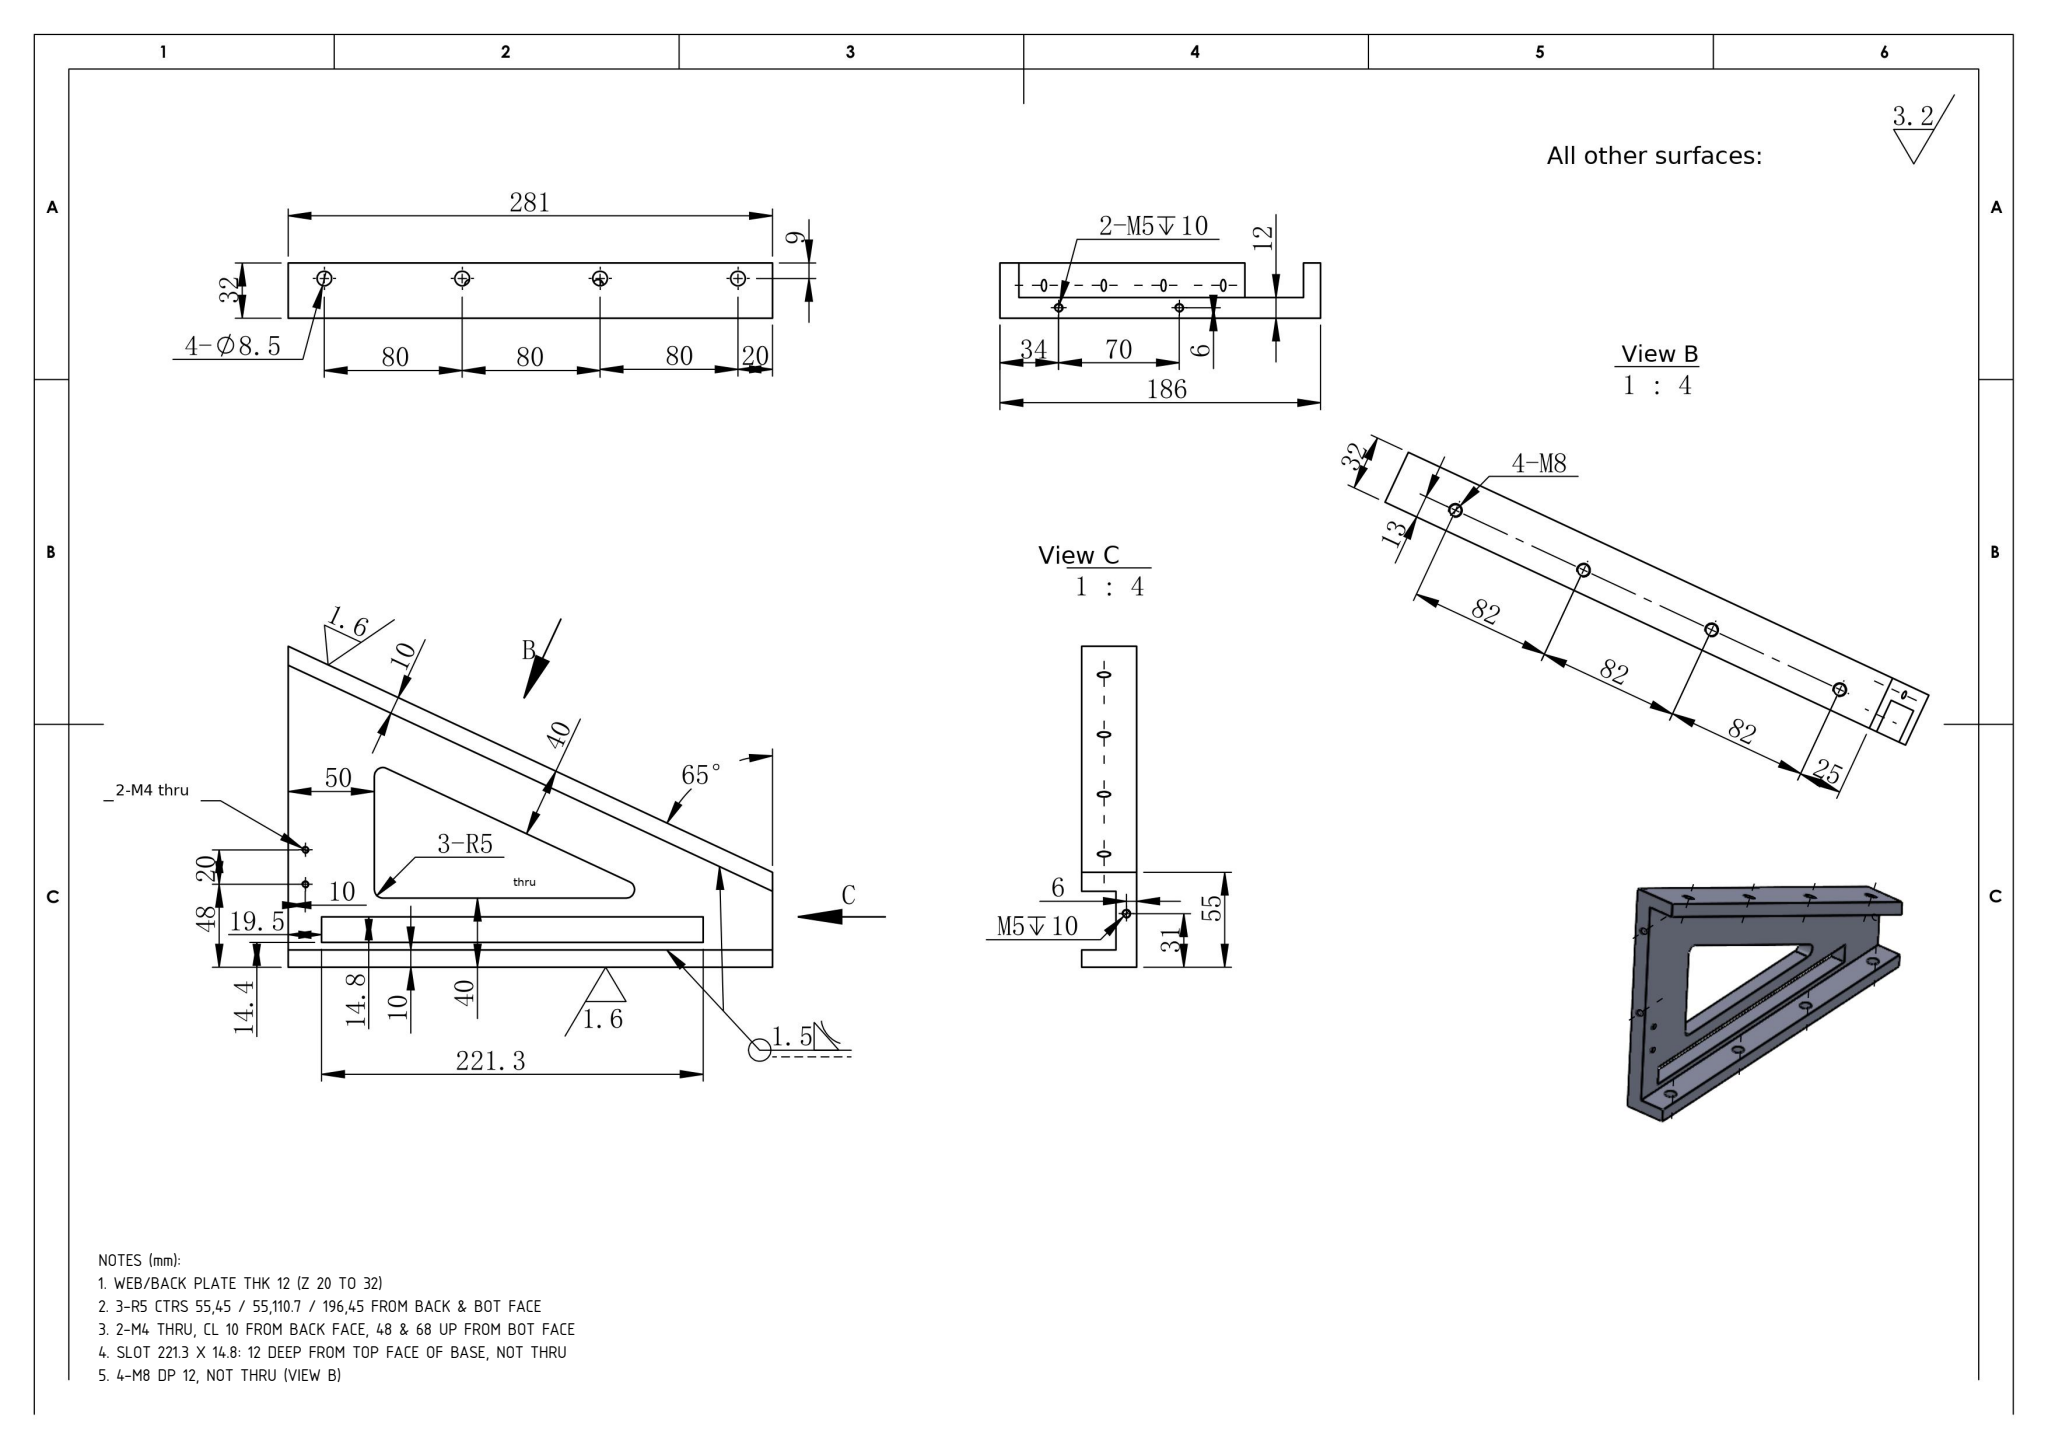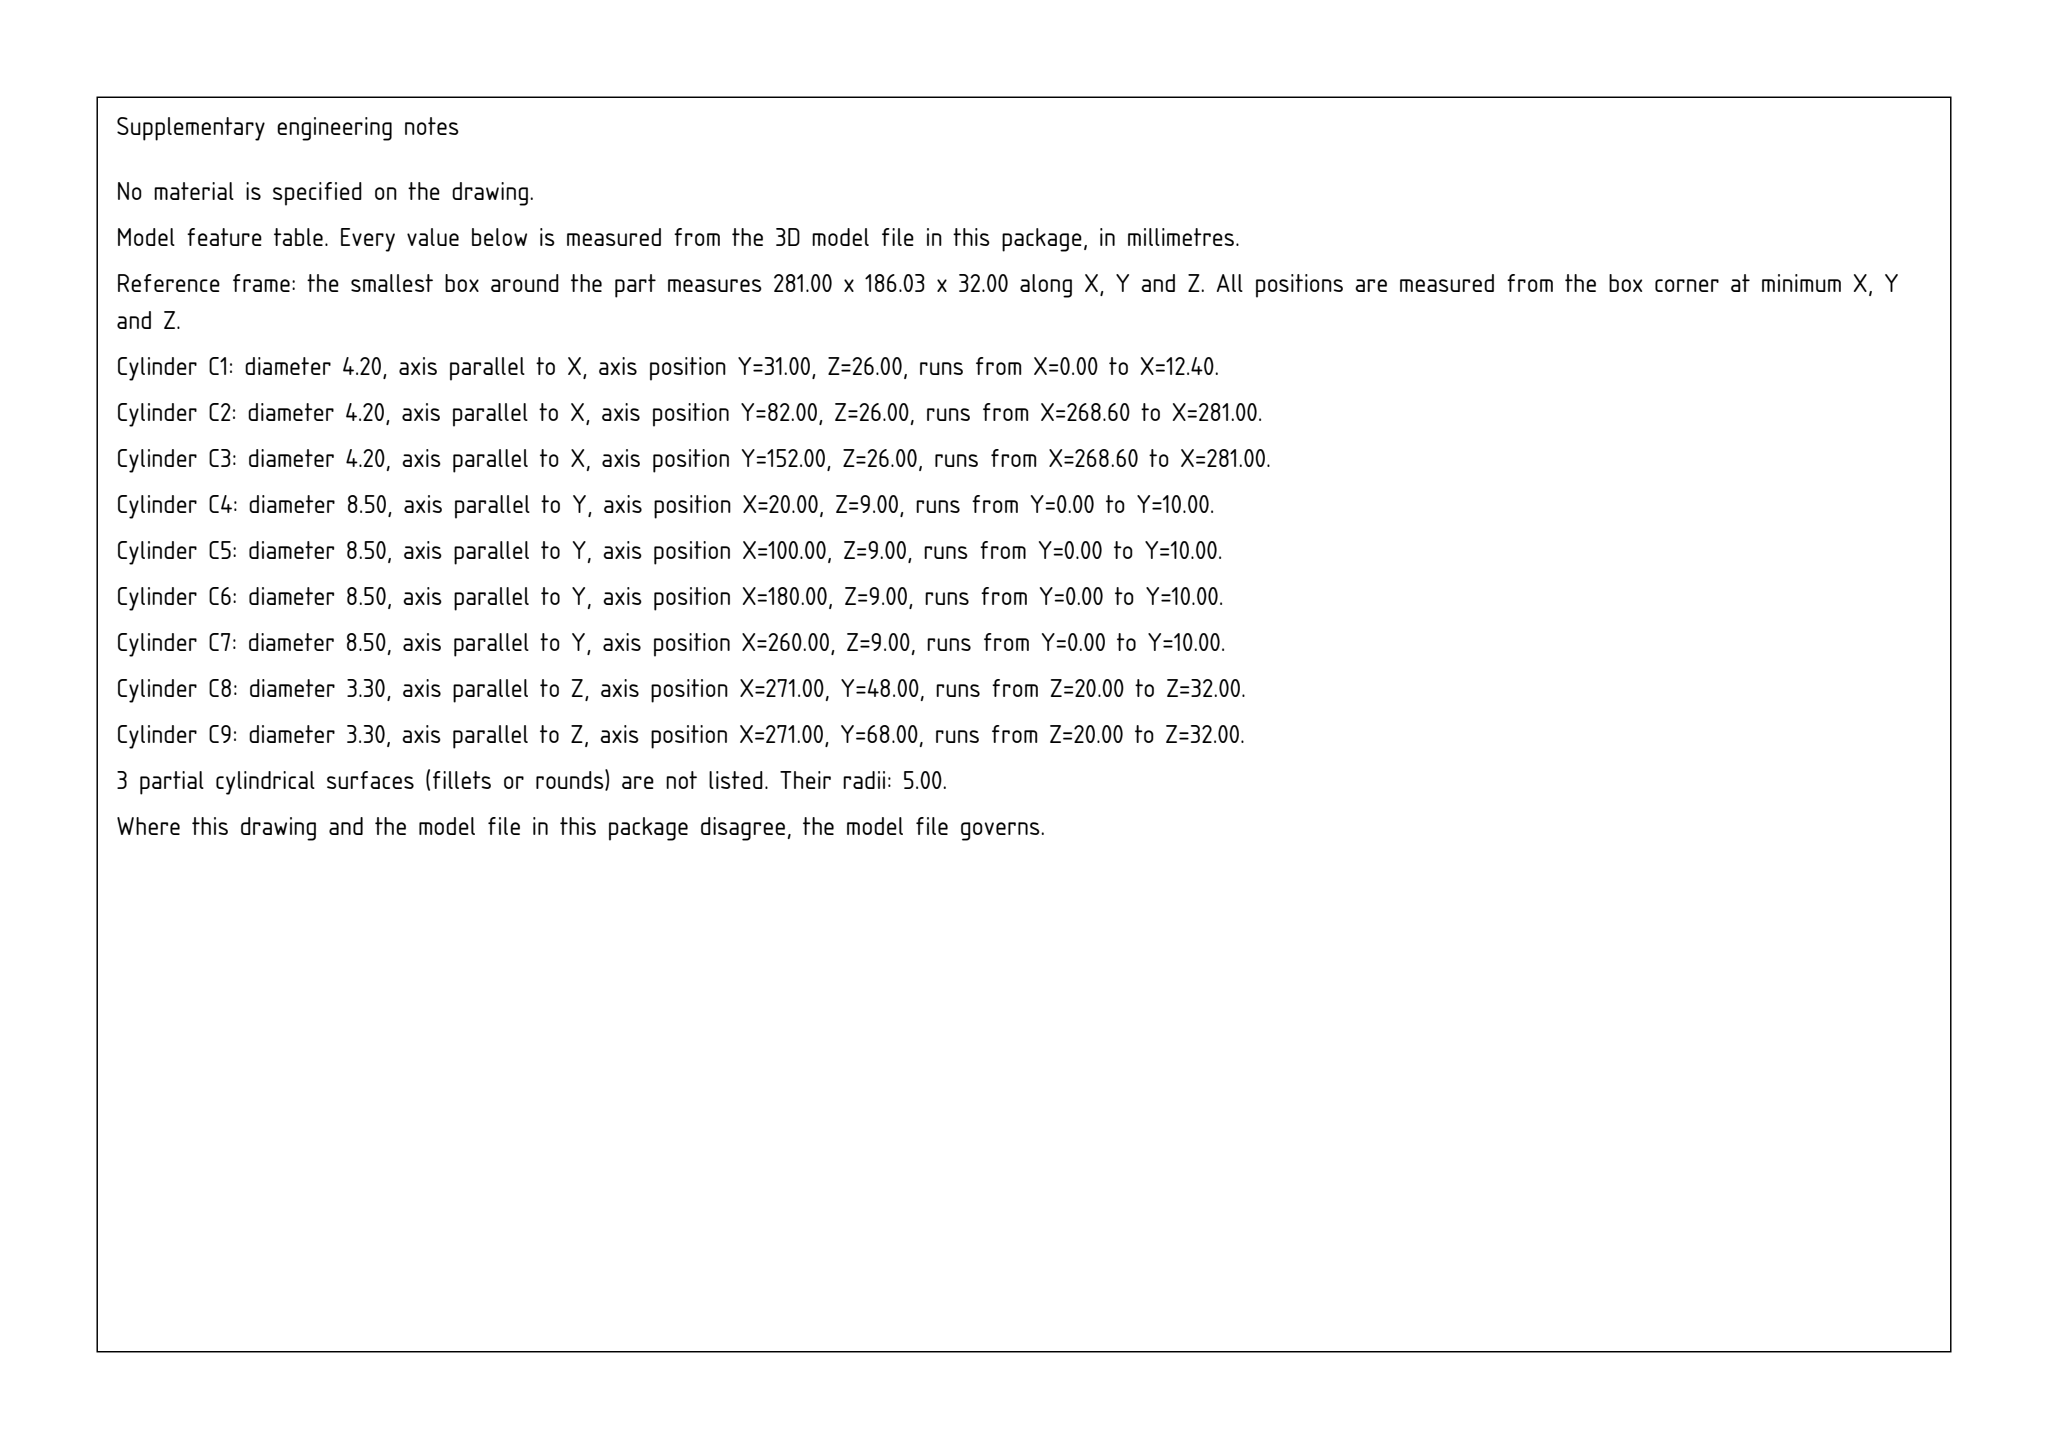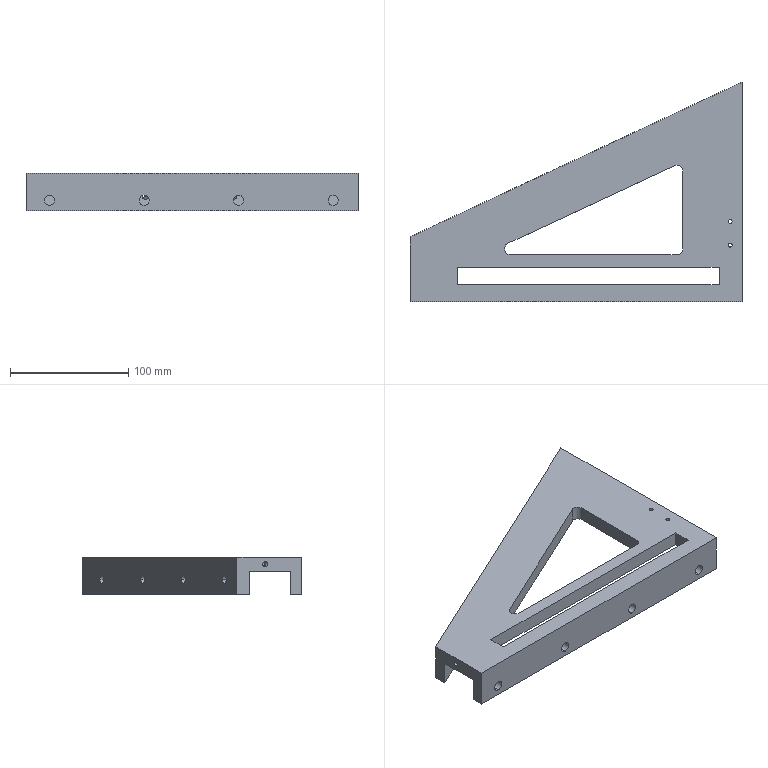Part | SolidWorks | mm | 1 solid | 53 faces | box 281 x 186.03 x 32 mm | volume 402540 mm3 | cylinder 30 | plane 17 | cone 6 | commonest cylinder face diameters 8.5 x8 6.8 x8 4.2 x6 3.3 x4 10 x4
Drawing notes:
WEB/BACK PLATE THK 12 (Z 20 TO 32) | from the solid: axis_planes z=20 & z=32; M4 holes len 12.0; R5 pocket cyls len 12.0
3-R5 CTRS 55,45 / 55,110.7 / 196,45 FROM BACK & BOT FACE | from the solid: Ø10 z-axis cyls at (85.03,45),(226,45),(226,110.73); 281-226=55, 281-85.03=195.97
2-M4 THRU, CL 10 FROM BACK FACE, 48 & 68 UP FROM BOT FACE | from the solid: Ø3.3 z-axis holes at x=271 (281-271=10), y=48 and y=68, thru 12
SLOT 221.3 X 14.8: 12 DEEP FROM TOP FACE OF BASE, NOT THRU | from the solid: Slot faces x 40.23-261.54 (221.31), y 14.35-29.16 (14.81); z planes 32 (top) to 20 => 12 deep, bbox z 0-32
4-M8 DP 12, NOT THRU (VIEW B) | from the solid: 4x dia 6.8 cyl, axis y, length 11.94, z=13, at x 22.66/96.97/171.29/245.61 (82 pitch)